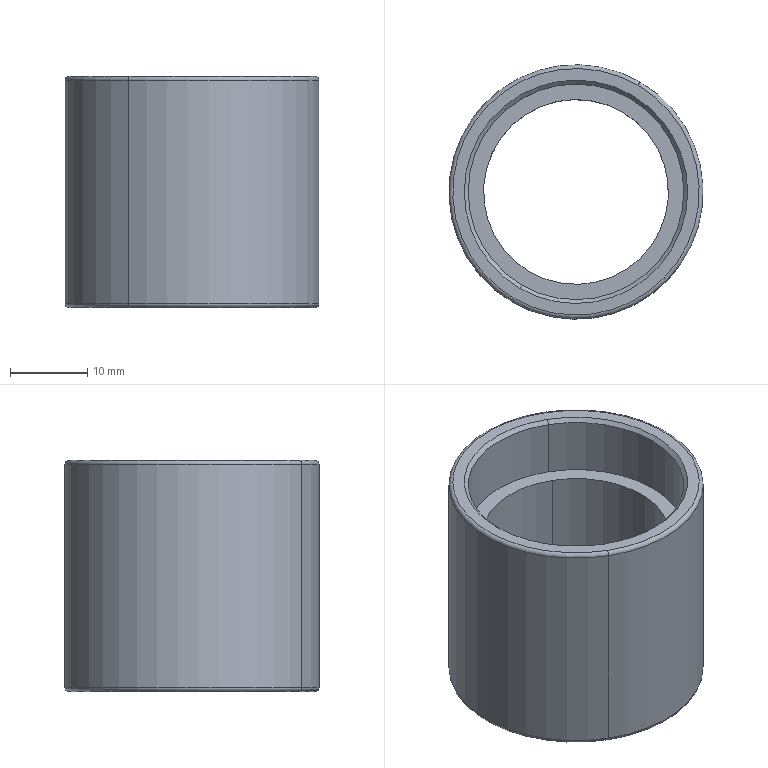Component | SolidWorks | 8TC-A15004-D0-16A-1 | 1 solid | 20 faces | box 33 x 33 x 30 mm | volume 9440 mm3 | cylinder 8 | cone 4 | torus 4 | plane 4 | commonest cylinder face diameters 28 x4 33 x2 24 x2 | material #45
build123d program:
from build123d import *

# Parameters (mm, degrees)
FILLET1_R     = 0.5
CHAMFER1_SIZE = 0.5


with BuildPart() as part:
    # Sketch1 → Revolve1 (revolve)
    with BuildSketch(Plane.XY):
        Polygon((-30, 14), (-30, 16.5), (0, 16.5), (0, 14), (-8, 14), (-8, 12), (-22, 12), (-22, 14), align=None)
    revolve(axis=Axis((0, 0, 0), (-1, 0, 0)))

    # Fillet1
    fillet1_edges = [part.edges().sort_by_distance(p)[0] for p in [
        (0, -16.5, 0),
        (-30, -16.5, 0),
    ]]
    fillet(fillet1_edges, radius=FILLET1_R)

    # Chamfer1
    chamfer1_edges = [part.edges().sort_by_distance(p)[0] for p in [
        (0, -14, 0),
        (-30, -14, 0),
    ]]
    chamfer(chamfer1_edges, length=CHAMFER1_SIZE)


solid = part.part

# Placed as in the assembly
solid = solid.moved(Location((29.5, 189.5, 131), (0, 90, 0)))
STEP:
#1=COLOUR_RGB('',0.7922,0.8196,0.9333);
#2=FILL_AREA_STYLE_COLOUR('',#1);
#3=FILL_AREA_STYLE('',(#2));
#4=SURFACE_STYLE_FILL_AREA(#3);
#5=SURFACE_SIDE_STYLE('',(#4));
#6=SURFACE_STYLE_USAGE(.BOTH.,#5);
#7=PRESENTATION_STYLE_ASSIGNMENT((#6));
#8=CARTESIAN_POINT('',(0.8841,6.984,6.319));
#9=VERTEX_POINT('',#8);
#10=CARTESIAN_POINT('',(1.439,7.937,6.319));
#11=VERTEX_POINT('',#10);
#12=CARTESIAN_POINT('',(1.161,7.461,6.319));
#13=DIRECTION('',(-0.,-0.,1.));
#14=DIRECTION('',(0.5031,0.8642,0.));
#15=AXIS2_PLACEMENT_3D('',#12,#13,#14);
#16=CIRCLE('',#15,0.5512);
#17=EDGE_CURVE('',#9,#11,#16,.T.);
#18=ORIENTED_EDGE('',*,*,#17,.F.);
#19=CARTESIAN_POINT('',(0.8742,6.967,6.339));
#20=VERTEX_POINT('',#19);
#21=CARTESIAN_POINT('',(0.8841,6.984,6.319));
#22=DIRECTION('',(-0.3558,-0.6111,0.7071));
#23=VECTOR('',#22,39.37);
#24=LINE('',#21,#23);
#25=EDGE_CURVE('',#9,#20,#24,.T.);
#26=ORIENTED_EDGE('',*,*,#25,.T.);
#27=CARTESIAN_POINT('',(1.449,7.954,6.339));
#28=VERTEX_POINT('',#27);
#29=CARTESIAN_POINT('',(1.161,7.461,6.339));
#30=DIRECTION('',(0.,0.,-1.));
#31=DIRECTION('',(0.5031,0.8642,0.));
#32=AXIS2_PLACEMENT_3D('',#29,#30,#31);
#33=CIRCLE('',#32,0.5709);
#34=EDGE_CURVE('',#28,#20,#33,.T.);
#35=ORIENTED_EDGE('',*,*,#34,.F.);
#36=CARTESIAN_POINT('',(1.439,7.937,6.319));
#37=DIRECTION('',(0.3558,0.6111,0.7071));
#38=VECTOR('',#37,39.37);
#39=LINE('',#36,#38);
#40=EDGE_CURVE('',#11,#28,#39,.T.);
#41=ORIENTED_EDGE('',*,*,#40,.F.);
#42=EDGE_LOOP('',(#18,#26,#35,#41));
#43=FACE_OUTER_BOUND('',#42,.T.);
#44=CARTESIAN_POINT('',(1.161,7.461,6.319));
#45=DIRECTION('',(-0.,-0.,1.));
#46=DIRECTION('',(0.5031,0.8642,0.));
#47=AXIS2_PLACEMENT_3D('',#44,#45,#46);
#48=CONICAL_SURFACE('',#47,0.5512,0.7854);
#49=ADVANCED_FACE('',(#43),#48,.F.);
#50=CARTESIAN_POINT('',(1.439,7.937,5.177));
#51=VERTEX_POINT('',#50);
#52=CARTESIAN_POINT('',(0.8841,6.984,5.177));
#53=VERTEX_POINT('',#52);
#54=CARTESIAN_POINT('',(1.161,7.461,5.177));
#55=DIRECTION('',(0.,0.,-1.));
#56=DIRECTION('',(-0.5031,-0.8642,0.));
#57=AXIS2_PLACEMENT_3D('',#54,#55,#56);
#58=CIRCLE('',#57,0.5512);
#59=EDGE_CURVE('',#51,#53,#58,.T.);
#60=ORIENTED_EDGE('',*,*,#59,.F.);
#61=CARTESIAN_POINT('',(1.449,7.954,5.157));
#62=VERTEX_POINT('',#61);
#63=CARTESIAN_POINT('',(1.449,7.954,5.157));
#64=DIRECTION('',(0.3558,0.6111,-0.7071));
#65=VECTOR('',#64,39.37);
#66=LINE('',#63,#65);
#67=EDGE_CURVE('',#51,#62,#66,.T.);
#68=ORIENTED_EDGE('',*,*,#67,.T.);
#69=CARTESIAN_POINT('',(0.8742,6.967,5.157));
#70=VERTEX_POINT('',#69);
#71=CARTESIAN_POINT('',(1.161,7.461,5.157));
#72=DIRECTION('',(-0.,-0.,1.));
#73=DIRECTION('',(-0.5031,-0.8642,0.));
#74=AXIS2_PLACEMENT_3D('',#71,#72,#73);
#75=CIRCLE('',#74,0.5709);
#76=EDGE_CURVE('',#70,#62,#75,.T.);
#77=ORIENTED_EDGE('',*,*,#76,.F.);
#78=CARTESIAN_POINT('',(0.8742,6.967,5.157));
#79=DIRECTION('',(-0.3558,-0.6111,-0.7071));
#80=VECTOR('',#79,39.37);
#81=LINE('',#78,#80);
#82=EDGE_CURVE('',#53,#70,#81,.T.);
#83=ORIENTED_EDGE('',*,*,#82,.F.);
#84=EDGE_LOOP('',(#60,#68,#77,#83));
#85=FACE_OUTER_BOUND('',#84,.T.);
#86=CARTESIAN_POINT('',(1.161,7.461,5.157));
#87=DIRECTION('',(0.,0.,-1.));
#88=DIRECTION('',(-0.5031,-0.8642,0.));
#89=AXIS2_PLACEMENT_3D('',#86,#87,#88);
#90=CONICAL_SURFACE('',#89,0.5709,0.7854);
#91=ADVANCED_FACE('',(#85),#90,.F.);
#92=CARTESIAN_POINT('',(0.8346,6.899,6.319));
#93=VERTEX_POINT('',#92);
#94=CARTESIAN_POINT('',(1.488,8.022,6.319));
#95=VERTEX_POINT('',#94);
#96=CARTESIAN_POINT('',(1.161,7.461,6.319));
#97=DIRECTION('',(0.,0.,-1.));
#98=DIRECTION('',(0.5031,0.8642,0.));
#99=AXIS2_PLACEMENT_3D('',#96,#97,#98);
#100=CIRCLE('',#99,0.6496);
#101=EDGE_CURVE('',#93,#95,#100,.T.);
#102=ORIENTED_EDGE('',*,*,#101,.F.);
#103=CARTESIAN_POINT('',(0.8445,6.916,6.339));
#104=VERTEX_POINT('',#103);
#105=CARTESIAN_POINT('',(0.8445,6.916,6.319));
#106=DIRECTION('',(-0.8642,0.5031,0.));
#107=DIRECTION('',(-0.5031,-0.8642,0.));
#108=AXIS2_PLACEMENT_3D('',#105,#106,#107);
#109=CIRCLE('',#108,0.01969);
#110=EDGE_CURVE('',#93,#104,#109,.T.);
#111=ORIENTED_EDGE('',*,*,#110,.T.);
#112=CARTESIAN_POINT('',(1.478,8.005,6.339));
#113=VERTEX_POINT('',#112);
#114=CARTESIAN_POINT('',(1.161,7.461,6.339));
#115=DIRECTION('',(-0.,-0.,1.));
#116=DIRECTION('',(0.5031,0.8642,0.));
#117=AXIS2_PLACEMENT_3D('',#114,#115,#116);
#118=CIRCLE('',#117,0.6299);
#119=EDGE_CURVE('',#113,#104,#118,.T.);
#120=ORIENTED_EDGE('',*,*,#119,.F.);
#121=CARTESIAN_POINT('',(1.478,8.005,6.319));
#122=DIRECTION('',(0.8642,-0.5031,-0.));
#123=DIRECTION('',(0.5031,0.8642,0.));
#124=AXIS2_PLACEMENT_3D('',#121,#122,#123);
#125=CIRCLE('',#124,0.01969);
#126=EDGE_CURVE('',#95,#113,#125,.T.);
#127=ORIENTED_EDGE('',*,*,#126,.F.);
#128=EDGE_LOOP('',(#102,#111,#120,#127));
#129=FACE_OUTER_BOUND('',#128,.T.);
#130=CARTESIAN_POINT('',(1.161,7.461,6.319));
#131=DIRECTION('',(-0.,-0.,1.));
#132=DIRECTION('',(0.5031,0.8642,0.));
#133=AXIS2_PLACEMENT_3D('',#130,#131,#132);
#134=TOROIDAL_SURFACE('',#133,0.6299,0.01969);
#135=ADVANCED_FACE('',(#129),#134,.T.);
#136=CARTESIAN_POINT('',(1.488,8.022,5.177));
#137=VERTEX_POINT('',#136);
#138=CARTESIAN_POINT('',(0.8346,6.899,5.177));
#139=VERTEX_POINT('',#138);
#140=CARTESIAN_POINT('',(1.161,7.461,5.177));
#141=DIRECTION('',(-0.,-0.,1.));
#142=DIRECTION('',(-0.5031,-0.8642,0.));
#143=AXIS2_PLACEMENT_3D('',#140,#141,#142);
#144=CIRCLE('',#143,0.6496);
#145=EDGE_CURVE('',#137,#139,#144,.T.);
#146=ORIENTED_EDGE('',*,*,#145,.F.);
#147=CARTESIAN_POINT('',(1.478,8.005,5.157));
#148=VERTEX_POINT('',#147);
#149=CARTESIAN_POINT('',(1.478,8.005,5.177));
#150=DIRECTION('',(-0.8642,0.5031,0.));
#151=DIRECTION('',(-0.5031,-0.8642,0.));
#152=AXIS2_PLACEMENT_3D('',#149,#150,#151);
#153=CIRCLE('',#152,0.01969);
#154=EDGE_CURVE('',#137,#148,#153,.T.);
#155=ORIENTED_EDGE('',*,*,#154,.T.);
#156=CARTESIAN_POINT('',(0.8445,6.916,5.157));
#157=VERTEX_POINT('',#156);
#158=CARTESIAN_POINT('',(1.161,7.461,5.157));
#159=DIRECTION('',(0.,0.,-1.));
#160=DIRECTION('',(-0.5031,-0.8642,0.));
#161=AXIS2_PLACEMENT_3D('',#158,#159,#160);
#162=CIRCLE('',#161,0.6299);
#163=EDGE_CURVE('',#157,#148,#162,.T.);
#164=ORIENTED_EDGE('',*,*,#163,.F.);
#165=CARTESIAN_POINT('',(0.8445,6.916,5.177));
#166=DIRECTION('',(0.8642,-0.5031,-0.));
#167=DIRECTION('',(0.5031,0.8642,0.));
#168=AXIS2_PLACEMENT_3D('',#165,#166,#167);
#169=CIRCLE('',#168,0.01969);
#170=EDGE_CURVE('',#139,#157,#169,.T.);
#171=ORIENTED_EDGE('',*,*,#170,.F.);
#172=EDGE_LOOP('',(#146,#155,#164,#171));
#173=FACE_OUTER_BOUND('',#172,.T.);
#174=CARTESIAN_POINT('',(1.161,7.461,5.177));
#175=DIRECTION('',(0.,0.,-1.));
#176=DIRECTION('',(-0.5031,-0.8642,-0.));
#177=AXIS2_PLACEMENT_3D('',#174,#175,#176);
#178=TOROIDAL_SURFACE('',#177,0.6299,0.01969);
#179=ADVANCED_FACE('',(#173),#178,.T.);
#180=CARTESIAN_POINT('',(0.8841,6.984,6.024));
#181=VERTEX_POINT('',#180);
#182=CARTESIAN_POINT('',(1.439,7.937,6.024));
#183=VERTEX_POINT('',#182);
#184=CARTESIAN_POINT('',(1.161,7.461,6.024));
#185=DIRECTION('',(-0.,-0.,1.));
#186=DIRECTION('',(0.5031,0.8642,0.));
#187=AXIS2_PLACEMENT_3D('',#184,#185,#186);
#188=CIRCLE('',#187,0.5512);
#189=EDGE_CURVE('',#181,#183,#188,.T.);
#190=ORIENTED_EDGE('',*,*,#189,.F.);
#191=CARTESIAN_POINT('',(0.8841,6.984,6.339));
#192=DIRECTION('',(-0.,-0.,1.));
#193=VECTOR('',#192,39.37);
#194=LINE('',#191,#193);
#195=EDGE_CURVE('',#181,#9,#194,.T.);
#196=ORIENTED_EDGE('',*,*,#195,.T.);
#197=ORIENTED_EDGE('',*,*,#17,.T.);
#198=CARTESIAN_POINT('',(1.439,7.937,6.339));
#199=DIRECTION('',(-0.,-0.,1.));
#200=VECTOR('',#199,39.37);
#201=LINE('',#198,#200);
#202=EDGE_CURVE('',#183,#11,#201,.T.);
#203=ORIENTED_EDGE('',*,*,#202,.F.);
#204=EDGE_LOOP('',(#190,#196,#197,#203));
#205=FACE_OUTER_BOUND('',#204,.T.);
#206=CARTESIAN_POINT('',(1.161,7.461,6.339));
#207=DIRECTION('',(-0.,-0.,1.));
#208=DIRECTION('',(0.5031,0.8642,0.));
#209=AXIS2_PLACEMENT_3D('',#206,#207,#208);
#210=CYLINDRICAL_SURFACE('',#209,0.5512);
#211=ADVANCED_FACE('',(#205),#210,.F.);
#212=ORIENTED_EDGE('',*,*,#145,.T.);
#213=CARTESIAN_POINT('',(0.8346,6.899,6.339));
#214=DIRECTION('',(-0.,-0.,1.));
#215=VECTOR('',#214,39.37);
#216=LINE('',#213,#215);
#217=EDGE_CURVE('',#139,#93,#216,.T.);
#218=ORIENTED_EDGE('',*,*,#217,.T.);
#219=ORIENTED_EDGE('',*,*,#101,.T.);
#220=CARTESIAN_POINT('',(1.488,8.022,6.339));
#221=DIRECTION('',(-0.,-0.,1.));
#222=VECTOR('',#221,39.37);
#223=LINE('',#220,#222);
#224=EDGE_CURVE('',#137,#95,#223,.T.);
#225=ORIENTED_EDGE('',*,*,#224,.F.);
#226=EDGE_LOOP('',(#212,#218,#219,#225));
#227=FACE_OUTER_BOUND('',#226,.T.);
#228=CARTESIAN_POINT('',(1.161,7.461,6.339));
#229=DIRECTION('',(-0.,-0.,1.));
#230=DIRECTION('',(0.5031,0.8642,0.));
#231=AXIS2_PLACEMENT_3D('',#228,#229,#230);
#232=CYLINDRICAL_SURFACE('',#231,0.6496);
#233=ADVANCED_FACE('',(#227),#232,.T.);
#234=ORIENTED_EDGE('',*,*,#59,.T.);
#235=CARTESIAN_POINT('',(0.8841,6.984,5.472));
#236=VERTEX_POINT('',#235);
#237=CARTESIAN_POINT('',(0.8841,6.984,6.339));
#238=DIRECTION('',(-0.,-0.,1.));
#239=VECTOR('',#238,39.37);
#240=LINE('',#237,#239);
#241=EDGE_CURVE('',#53,#236,#240,.T.);
#242=ORIENTED_EDGE('',*,*,#241,.T.);
#243=CARTESIAN_POINT('',(1.439,7.937,5.472));
#244=VERTEX_POINT('',#243);
#245=CARTESIAN_POINT('',(1.161,7.461,5.472));
#246=DIRECTION('',(-0.,-0.,1.));
#247=DIRECTION('',(0.5031,0.8642,0.));
#248=AXIS2_PLACEMENT_3D('',#245,#246,#247);
#249=CIRCLE('',#248,0.5512);
#250=EDGE_CURVE('',#236,#244,#249,.T.);
#251=ORIENTED_EDGE('',*,*,#250,.T.);
#252=CARTESIAN_POINT('',(1.439,7.937,6.339));
#253=DIRECTION('',(-0.,-0.,1.));
#254=VECTOR('',#253,39.37);
#255=LINE('',#252,#254);
#256=EDGE_CURVE('',#51,#244,#255,.T.);
#257=ORIENTED_EDGE('',*,*,#256,.F.);
#258=EDGE_LOOP('',(#234,#242,#251,#257));
#259=FACE_OUTER_BOUND('',#258,.T.);
#260=CARTESIAN_POINT('',(1.161,7.461,6.339));
#261=DIRECTION('',(-0.,-0.,1.));
#262=DIRECTION('',(0.5031,0.8642,0.));
#263=AXIS2_PLACEMENT_3D('',#260,#261,#262);
#264=CYLINDRICAL_SURFACE('',#263,0.5512);
#265=ADVANCED_FACE('',(#259),#264,.F.);
#266=CARTESIAN_POINT('',(0.9237,7.052,5.472));
#267=VERTEX_POINT('',#266);
#268=CARTESIAN_POINT('',(1.399,7.869,5.472));
#269=VERTEX_POINT('',#268);
#270=CARTESIAN_POINT('',(1.161,7.461,5.472));
#271=DIRECTION('',(-0.,-0.,1.));
#272=DIRECTION('',(0.5031,0.8642,0.));
#273=AXIS2_PLACEMENT_3D('',#270,#271,#272);
#274=CIRCLE('',#273,0.4724);
#275=EDGE_CURVE('',#267,#269,#274,.T.);
#276=ORIENTED_EDGE('',*,*,#275,.F.);
#277=CARTESIAN_POINT('',(0.9237,7.052,6.024));
#278=VERTEX_POINT('',#277);
#279=CARTESIAN_POINT('',(0.9237,7.052,6.339));
#280=DIRECTION('',(-0.,-0.,1.));
#281=VECTOR('',#280,39.37);
#282=LINE('',#279,#281);
#283=EDGE_CURVE('',#267,#278,#282,.T.);
#284=ORIENTED_EDGE('',*,*,#283,.T.);
#285=CARTESIAN_POINT('',(1.399,7.869,6.024));
#286=VERTEX_POINT('',#285);
#287=CARTESIAN_POINT('',(1.161,7.461,6.024));
#288=DIRECTION('',(-0.,-0.,1.));
#289=DIRECTION('',(0.5031,0.8642,0.));
#290=AXIS2_PLACEMENT_3D('',#287,#288,#289);
#291=CIRCLE('',#290,0.4724);
#292=EDGE_CURVE('',#278,#286,#291,.T.);
#293=ORIENTED_EDGE('',*,*,#292,.T.);
#294=CARTESIAN_POINT('',(1.399,7.869,6.339));
#295=DIRECTION('',(-0.,-0.,1.));
#296=VECTOR('',#295,39.37);
#297=LINE('',#294,#296);
#298=EDGE_CURVE('',#269,#286,#297,.T.);
#299=ORIENTED_EDGE('',*,*,#298,.F.);
#300=EDGE_LOOP('',(#276,#284,#293,#299));
#301=FACE_OUTER_BOUND('',#300,.T.);
#302=CARTESIAN_POINT('',(1.161,7.461,6.339));
#303=DIRECTION('',(-0.,-0.,1.));
#304=DIRECTION('',(0.5031,0.8642,0.));
#305=AXIS2_PLACEMENT_3D('',#302,#303,#304);
#306=CYLINDRICAL_SURFACE('',#305,0.4724);
#307=ADVANCED_FACE('',(#301),#306,.F.);
#308=ORIENTED_EDGE('',*,*,#283,.F.);
#309=CARTESIAN_POINT('',(1.161,7.461,5.472));
#310=DIRECTION('',(-0.,-0.,1.));
#311=DIRECTION('',(0.5031,0.8642,0.));
#312=AXIS2_PLACEMENT_3D('',#309,#310,#311);
#313=CIRCLE('',#312,0.4724);
#314=EDGE_CURVE('',#269,#267,#313,.T.);
#315=ORIENTED_EDGE('',*,*,#314,.F.);
#316=ORIENTED_EDGE('',*,*,#298,.T.);
#317=CARTESIAN_POINT('',(1.161,7.461,6.024));
#318=DIRECTION('',(-0.,-0.,1.));
#319=DIRECTION('',(0.5031,0.8642,0.));
#320=AXIS2_PLACEMENT_3D('',#317,#318,#319);
#321=CIRCLE('',#320,0.4724);
#322=EDGE_CURVE('',#286,#278,#321,.T.);
#323=ORIENTED_EDGE('',*,*,#322,.T.);
#324=EDGE_LOOP('',(#308,#315,#316,#323));
#325=FACE_OUTER_BOUND('',#324,.T.);
#326=CARTESIAN_POINT('',(1.161,7.461,6.339));
#327=DIRECTION('',(-0.,-0.,1.));
#328=DIRECTION('',(0.5031,0.8642,0.));
#329=AXIS2_PLACEMENT_3D('',#326,#327,#328);
#330=CYLINDRICAL_SURFACE('',#329,0.4724);
#331=ADVANCED_FACE('',(#325),#330,.F.);
#332=ORIENTED_EDGE('',*,*,#314,.T.);
#333=ORIENTED_EDGE('',*,*,#275,.T.);
#334=EDGE_LOOP('',(#332,#333));
#335=FACE_BOUND('',#334,.T.);
#336=CARTESIAN_POINT('',(1.161,7.461,5.472));
#337=DIRECTION('',(-0.,-0.,1.));
#338=DIRECTION('',(0.5031,0.8642,0.));
#339=AXIS2_PLACEMENT_3D('',#336,#337,#338);
#340=CIRCLE('',#339,0.5512);
#341=EDGE_CURVE('',#244,#236,#340,.T.);
#342=ORIENTED_EDGE('',*,*,#341,.F.);
#343=ORIENTED_EDGE('',*,*,#250,.F.);
#344=EDGE_LOOP('',(#342,#343));
#345=FACE_OUTER_BOUND('',#344,.T.);
#346=CARTESIAN_POINT('',(1.399,7.869,5.472));
#347=DIRECTION('',(0.,0.,-1.));
#348=DIRECTION('',(-0.5031,-0.8642,-0.));
#349=AXIS2_PLACEMENT_3D('',#346,#347,#348);
#350=PLANE('',#349);
#351=ADVANCED_FACE('',(#335,#345),#350,.T.);
#352=ORIENTED_EDGE('',*,*,#241,.F.);
#353=CARTESIAN_POINT('',(1.161,7.461,5.177));
#354=DIRECTION('',(0.,0.,-1.));
#355=DIRECTION('',(-0.5031,-0.8642,0.));
#356=AXIS2_PLACEMENT_3D('',#353,#354,#355);
#357=CIRCLE('',#356,0.5512);
#358=EDGE_CURVE('',#53,#51,#357,.T.);
#359=ORIENTED_EDGE('',*,*,#358,.T.);
#360=ORIENTED_EDGE('',*,*,#256,.T.);
#361=ORIENTED_EDGE('',*,*,#341,.T.);
#362=EDGE_LOOP('',(#352,#359,#360,#361));
#363=FACE_OUTER_BOUND('',#362,.T.);
#364=CARTESIAN_POINT('',(1.161,7.461,6.339));
#365=DIRECTION('',(-0.,-0.,1.));
#366=DIRECTION('',(0.5031,0.8642,0.));
#367=AXIS2_PLACEMENT_3D('',#364,#365,#366);
#368=CYLINDRICAL_SURFACE('',#367,0.5512);
#369=ADVANCED_FACE('',(#363),#368,.F.);
#370=ORIENTED_EDGE('',*,*,#76,.T.);
#371=CARTESIAN_POINT('',(1.161,7.461,5.157));
#372=DIRECTION('',(-0.,-0.,1.));
#373=DIRECTION('',(-0.5031,-0.8642,0.));
#374=AXIS2_PLACEMENT_3D('',#371,#372,#373);
#375=CIRCLE('',#374,0.5709);
#376=EDGE_CURVE('',#62,#70,#375,.T.);
#377=ORIENTED_EDGE('',*,*,#376,.T.);
#378=EDGE_LOOP('',(#370,#377));
#379=FACE_BOUND('',#378,.T.);
#380=ORIENTED_EDGE('',*,*,#163,.T.);
#381=CARTESIAN_POINT('',(1.161,7.461,5.157));
#382=DIRECTION('',(0.,0.,-1.));
#383=DIRECTION('',(-0.5031,-0.8642,0.));
#384=AXIS2_PLACEMENT_3D('',#381,#382,#383);
#385=CIRCLE('',#384,0.6299);
#386=EDGE_CURVE('',#148,#157,#385,.T.);
#387=ORIENTED_EDGE('',*,*,#386,.T.);
#388=EDGE_LOOP('',(#380,#387));
#389=FACE_OUTER_BOUND('',#388,.T.);
#390=CARTESIAN_POINT('',(1.439,7.937,5.157));
#391=DIRECTION('',(0.,0.,-1.));
#392=DIRECTION('',(-0.5031,-0.8642,-0.));
#393=AXIS2_PLACEMENT_3D('',#390,#391,#392);
#394=PLANE('',#393);
#395=ADVANCED_FACE('',(#379,#389),#394,.T.);
#396=ORIENTED_EDGE('',*,*,#217,.F.);
#397=CARTESIAN_POINT('',(1.161,7.461,5.177));
#398=DIRECTION('',(-0.,-0.,1.));
#399=DIRECTION('',(-0.5031,-0.8642,0.));
#400=AXIS2_PLACEMENT_3D('',#397,#398,#399);
#401=CIRCLE('',#400,0.6496);
#402=EDGE_CURVE('',#139,#137,#401,.T.);
#403=ORIENTED_EDGE('',*,*,#402,.T.);
#404=ORIENTED_EDGE('',*,*,#224,.T.);
#405=CARTESIAN_POINT('',(1.161,7.461,6.319));
#406=DIRECTION('',(0.,0.,-1.));
#407=DIRECTION('',(0.5031,0.8642,0.));
#408=AXIS2_PLACEMENT_3D('',#405,#406,#407);
#409=CIRCLE('',#408,0.6496);
#410=EDGE_CURVE('',#95,#93,#409,.T.);
#411=ORIENTED_EDGE('',*,*,#410,.T.);
#412=EDGE_LOOP('',(#396,#403,#404,#411));
#413=FACE_OUTER_BOUND('',#412,.T.);
#414=CARTESIAN_POINT('',(1.161,7.461,6.339));
#415=DIRECTION('',(-0.,-0.,1.));
#416=DIRECTION('',(0.5031,0.8642,0.));
#417=AXIS2_PLACEMENT_3D('',#414,#415,#416);
#418=CYLINDRICAL_SURFACE('',#417,0.6496);
#419=ADVANCED_FACE('',(#413),#418,.T.);
#420=ORIENTED_EDGE('',*,*,#34,.T.);
#421=CARTESIAN_POINT('',(1.161,7.461,6.339));
#422=DIRECTION('',(0.,0.,-1.));
#423=DIRECTION('',(0.5031,0.8642,0.));
#424=AXIS2_PLACEMENT_3D('',#421,#422,#423);
#425=CIRCLE('',#424,0.5709);
#426=EDGE_CURVE('',#20,#28,#425,.T.);
#427=ORIENTED_EDGE('',*,*,#426,.T.);
#428=EDGE_LOOP('',(#420,#427));
#429=FACE_BOUND('',#428,.T.);
#430=ORIENTED_EDGE('',*,*,#119,.T.);
#431=CARTESIAN_POINT('',(1.161,7.461,6.339));
#432=DIRECTION('',(-0.,-0.,1.));
#433=DIRECTION('',(0.5031,0.8642,0.));
#434=AXIS2_PLACEMENT_3D('',#431,#432,#433);
#435=CIRCLE('',#434,0.6299);
#436=EDGE_CURVE('',#104,#113,#435,.T.);
#437=ORIENTED_EDGE('',*,*,#436,.T.);
#438=EDGE_LOOP('',(#430,#437));
#439=FACE_OUTER_BOUND('',#438,.T.);
#440=CARTESIAN_POINT('',(1.488,8.022,6.339));
#441=DIRECTION('',(-0.,-0.,1.));
#442=DIRECTION('',(0.5031,0.8642,0.));
#443=AXIS2_PLACEMENT_3D('',#440,#441,#442);
#444=PLANE('',#443);
#445=ADVANCED_FACE('',(#429,#439),#444,.T.);
#446=ORIENTED_EDGE('',*,*,#195,.F.);
#447=CARTESIAN_POINT('',(1.161,7.461,6.024));
#448=DIRECTION('',(-0.,-0.,1.));
#449=DIRECTION('',(0.5031,0.8642,0.));
#450=AXIS2_PLACEMENT_3D('',#447,#448,#449);
#451=CIRCLE('',#450,0.5512);
#452=EDGE_CURVE('',#183,#181,#451,.T.);
#453=ORIENTED_EDGE('',*,*,#452,.F.);
#454=ORIENTED_EDGE('',*,*,#202,.T.);
#455=CARTESIAN_POINT('',(1.161,7.461,6.319));
#456=DIRECTION('',(-0.,-0.,1.));
#457=DIRECTION('',(0.5031,0.8642,0.));
#458=AXIS2_PLACEMENT_3D('',#455,#456,#457);
#459=CIRCLE('',#458,0.5512);
#460=EDGE_CURVE('',#11,#9,#459,.T.);
#461=ORIENTED_EDGE('',*,*,#460,.T.);
#462=EDGE_LOOP('',(#446,#453,#454,#461));
#463=FACE_OUTER_BOUND('',#462,.T.);
#464=CARTESIAN_POINT('',(1.161,7.461,6.339));
#465=DIRECTION('',(-0.,-0.,1.));
#466=DIRECTION('',(0.5031,0.8642,0.));
#467=AXIS2_PLACEMENT_3D('',#464,#465,#466);
#468=CYLINDRICAL_SURFACE('',#467,0.5512);
#469=ADVANCED_FACE('',(#463),#468,.F.);
#470=ORIENTED_EDGE('',*,*,#452,.T.);
#471=ORIENTED_EDGE('',*,*,#189,.T.);
#472=EDGE_LOOP('',(#470,#471));
#473=FACE_OUTER_BOUND('',#472,.T.);
#474=ORIENTED_EDGE('',*,*,#322,.F.);
#475=ORIENTED_EDGE('',*,*,#292,.F.);
#476=EDGE_LOOP('',(#474,#475));
#477=FACE_BOUND('',#476,.T.);
#478=CARTESIAN_POINT('',(1.399,7.869,6.024));
#479=DIRECTION('',(-0.,-0.,1.));
#480=DIRECTION('',(0.5031,0.8642,0.));
#481=AXIS2_PLACEMENT_3D('',#478,#479,#480);
#482=PLANE('',#481);
#483=ADVANCED_FACE('',(#473,#477),#482,.T.);
#484=ORIENTED_EDGE('',*,*,#154,.F.);
#485=ORIENTED_EDGE('',*,*,#402,.F.);
#486=ORIENTED_EDGE('',*,*,#170,.T.);
#487=ORIENTED_EDGE('',*,*,#386,.F.);
#488=EDGE_LOOP('',(#484,#485,#486,#487));
#489=FACE_OUTER_BOUND('',#488,.T.);
#490=CARTESIAN_POINT('',(1.161,7.461,5.177));
#491=DIRECTION('',(0.,0.,-1.));
#492=DIRECTION('',(-0.5031,-0.8642,-0.));
#493=AXIS2_PLACEMENT_3D('',#490,#491,#492);
#494=TOROIDAL_SURFACE('',#493,0.6299,0.01969);
#495=ADVANCED_FACE('',(#489),#494,.T.);
#496=ORIENTED_EDGE('',*,*,#110,.F.);
#497=ORIENTED_EDGE('',*,*,#410,.F.);
#498=ORIENTED_EDGE('',*,*,#126,.T.);
#499=ORIENTED_EDGE('',*,*,#436,.F.);
#500=EDGE_LOOP('',(#496,#497,#498,#499));
#501=FACE_OUTER_BOUND('',#500,.T.);
#502=CARTESIAN_POINT('',(1.161,7.461,6.319));
#503=DIRECTION('',(-0.,-0.,1.));
#504=DIRECTION('',(0.5031,0.8642,0.));
#505=AXIS2_PLACEMENT_3D('',#502,#503,#504);
#506=TOROIDAL_SURFACE('',#505,0.6299,0.01969);
#507=ADVANCED_FACE('',(#501),#506,.T.);
#508=ORIENTED_EDGE('',*,*,#67,.F.);
#509=ORIENTED_EDGE('',*,*,#358,.F.);
#510=ORIENTED_EDGE('',*,*,#82,.T.);
#511=ORIENTED_EDGE('',*,*,#376,.F.);
#512=EDGE_LOOP('',(#508,#509,#510,#511));
#513=FACE_OUTER_BOUND('',#512,.T.);
#514=CARTESIAN_POINT('',(1.161,7.461,5.157));
#515=DIRECTION('',(0.,0.,-1.));
#516=DIRECTION('',(-0.5031,-0.8642,0.));
#517=AXIS2_PLACEMENT_3D('',#514,#515,#516);
#518=CONICAL_SURFACE('',#517,0.5709,0.7854);
#519=ADVANCED_FACE('',(#513),#518,.F.);
#520=ORIENTED_EDGE('',*,*,#25,.F.);
#521=ORIENTED_EDGE('',*,*,#460,.F.);
#522=ORIENTED_EDGE('',*,*,#40,.T.);
#523=ORIENTED_EDGE('',*,*,#426,.F.);
#524=EDGE_LOOP('',(#520,#521,#522,#523));
#525=FACE_OUTER_BOUND('',#524,.T.);
#526=CARTESIAN_POINT('',(1.161,7.461,6.319));
#527=DIRECTION('',(-0.,-0.,1.));
#528=DIRECTION('',(0.5031,0.8642,0.));
#529=AXIS2_PLACEMENT_3D('',#526,#527,#528);
#530=CONICAL_SURFACE('',#529,0.5512,0.7854);
#531=ADVANCED_FACE('',(#525),#530,.F.);
#532=CLOSED_SHELL('',(#49,#91,#135,#179,#211,#233,#265,#307,#331,#351,#369,#395,#419,#445,#469,#483,#495,#507,#519,#531));
#533=MANIFOLD_SOLID_BREP('',#532);
#534=STYLED_ITEM('',(#7),#533);
#535=(LENGTH_UNIT()NAMED_UNIT(*)SI_UNIT($,.METRE.));
#536=LENGTH_MEASURE_WITH_UNIT(LENGTH_MEASURE(0.0254),#535);
#537=DIMENSIONAL_EXPONENTS(1.,0.,0.,0.,0.,0.,0.);
#538=(CONVERSION_BASED_UNIT('',#536)LENGTH_UNIT()NAMED_UNIT(#537));
#539=UNCERTAINTY_MEASURE_WITH_UNIT(LENGTH_MEASURE(0.00001),#538,'','');
#540=(NAMED_UNIT(*)PLANE_ANGLE_UNIT()SI_UNIT($,.RADIAN.));
#541=(NAMED_UNIT(*)SI_UNIT($,.STERADIAN.)SOLID_ANGLE_UNIT());
#542=(GEOMETRIC_REPRESENTATION_CONTEXT(3)GLOBAL_UNCERTAINTY_ASSIGNED_CONTEXT((#539))GLOBAL_UNIT_ASSIGNED_CONTEXT((#538,#540,#541))REPRESENTATION_CONTEXT('',''));
#543=MECHANICAL_DESIGN_GEOMETRIC_PRESENTATION_REPRESENTATION('',(#534),#542);
#544=CARTESIAN_POINT('',(0.,0.,0.));
#545=DIRECTION('',(0.,0.,1.));
#546=DIRECTION('',(1.,0.,0.));
#547=AXIS2_PLACEMENT_3D('',#544,#545,#546);
#548=(LENGTH_UNIT()NAMED_UNIT(*)SI_UNIT($,.METRE.));
#549=LENGTH_MEASURE_WITH_UNIT(LENGTH_MEASURE(0.0254),#548);
#550=DIMENSIONAL_EXPONENTS(1.,0.,0.,0.,0.,0.,0.);
#551=(CONVERSION_BASED_UNIT('',#549)LENGTH_UNIT()NAMED_UNIT(#550));
#552=UNCERTAINTY_MEASURE_WITH_UNIT(LENGTH_MEASURE(0.00001),#551,'','');
#553=(NAMED_UNIT(*)PLANE_ANGLE_UNIT()SI_UNIT($,.RADIAN.));
#554=(NAMED_UNIT(*)SI_UNIT($,.STERADIAN.)SOLID_ANGLE_UNIT());
#555=(GEOMETRIC_REPRESENTATION_CONTEXT(3)GLOBAL_UNCERTAINTY_ASSIGNED_CONTEXT((#552))GLOBAL_UNIT_ASSIGNED_CONTEXT((#551,#553,#554))REPRESENTATION_CONTEXT('',''));
#556=ADVANCED_BREP_SHAPE_REPRESENTATION('',(#533,#547),#555);
#557=PRESENTATION_LAYER_ASSIGNMENT('','',(#534));